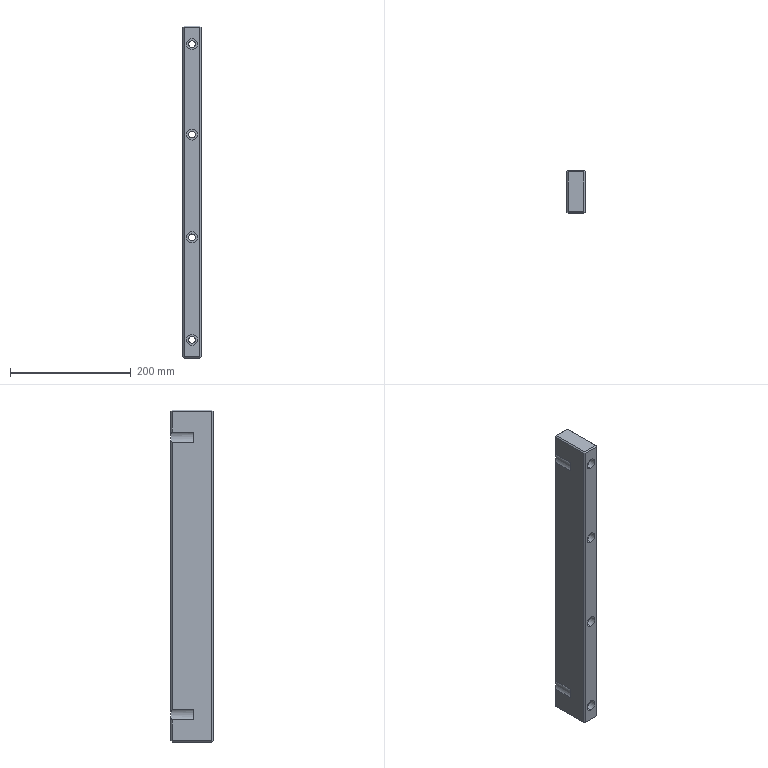Component | SolidWorks | LowerReinforcement(2)-1 | 1 solid | 56 faces | box 30 x 70 x 550 mm | volume 1111549 mm3 | plane 36 | cylinder 20 | commonest cylinder face diameters 18 x8 11 x8 26 x4
build123d program:
from build123d import *

# Parameters (mm, degrees)
SKETCH1_2_W                                      = 550
SKETCH1_2_H                                      = 30
BOSS_EXTRUDE1_DEPTH                              = 70
M10_HEX_SOCKET_HEAD_CAP_SCREW_CBORE1_D           = 11
M10_HEX_SOCKET_HEAD_CAP_SCREW_CBORE1_CBORE_D     = 18
M10_HEX_SOCKET_HEAD_CAP_SCREW_CBORE1_CBORE_DEPTH = 10.6
CHAMFER1_SIZE                                    = 2
CHAMFER2_SIZE                                    = 2
SKETCH1_R                                        = 13
GUIDEPOSTTENONRELIEF_DEPTH                       = 37


with BuildPart() as part:
    # Sketch1_2 → Boss-Extrude1 (new body)
    with BuildSketch(Plane.XY):
        with Locations((275, 15)):
            Rectangle(SKETCH1_2_W, SKETCH1_2_H)
    extrude(amount=BOSS_EXTRUDE1_DEPTH)

    # M10 Hex Socket Head Cap Screw CBORE1 (through all)
    with Locations(Plane.XY.offset(70)):
        with Locations((30, 15), (200, 15), (370, 15), (520, 15)):
            CounterBoreHole(M10_HEX_SOCKET_HEAD_CAP_SCREW_CBORE1_D / 2, M10_HEX_SOCKET_HEAD_CAP_SCREW_CBORE1_CBORE_D / 2, M10_HEX_SOCKET_HEAD_CAP_SCREW_CBORE1_CBORE_DEPTH)

    # Chamfer1
    chamfer1_edges = [part.edges().sort_by_distance(p)[0] for p in [
        (550, 15, 70),
        (275, 30, 70),
        (275, 30, 0),
        (550, 15, 0),
        (275, 0, 0),
        (0, 15, 0),
        (275, 0, 70),
        (0, 30, 35),
        (550, 30, 35),
        (550, 0, 35),
        (0, 0, 35),
    ]]
    chamfer(chamfer1_edges, length=CHAMFER1_SIZE)

    # Chamfer2
    chamfer2_edges = [part.edges().sort_by_distance(p)[0] for p in [
        (0, 15, 70),
    ]]
    chamfer(chamfer2_edges, length=CHAMFER2_SIZE)

    # Sketch1 → GuidePostTenonRelief (cut, symmetric)
    with BuildSketch(Plane.XY):
        with Locations((45, 40)):
            Circle(SKETCH1_R)
        with Locations((505, 40)):
            Circle(SKETCH1_R)
        with Locations((45, -10)):
            Circle(SKETCH1_R)
        with Locations((505, -10)):
            Circle(SKETCH1_R)
    extrude(amount=GUIDEPOSTTENONRELIEF_DEPTH, both=True, mode=Mode.SUBTRACT)


solid = part.part

# Placed as in the assembly
solid = solid.moved(Location((92.049, 277.323, -270), (90, 0, 90)))